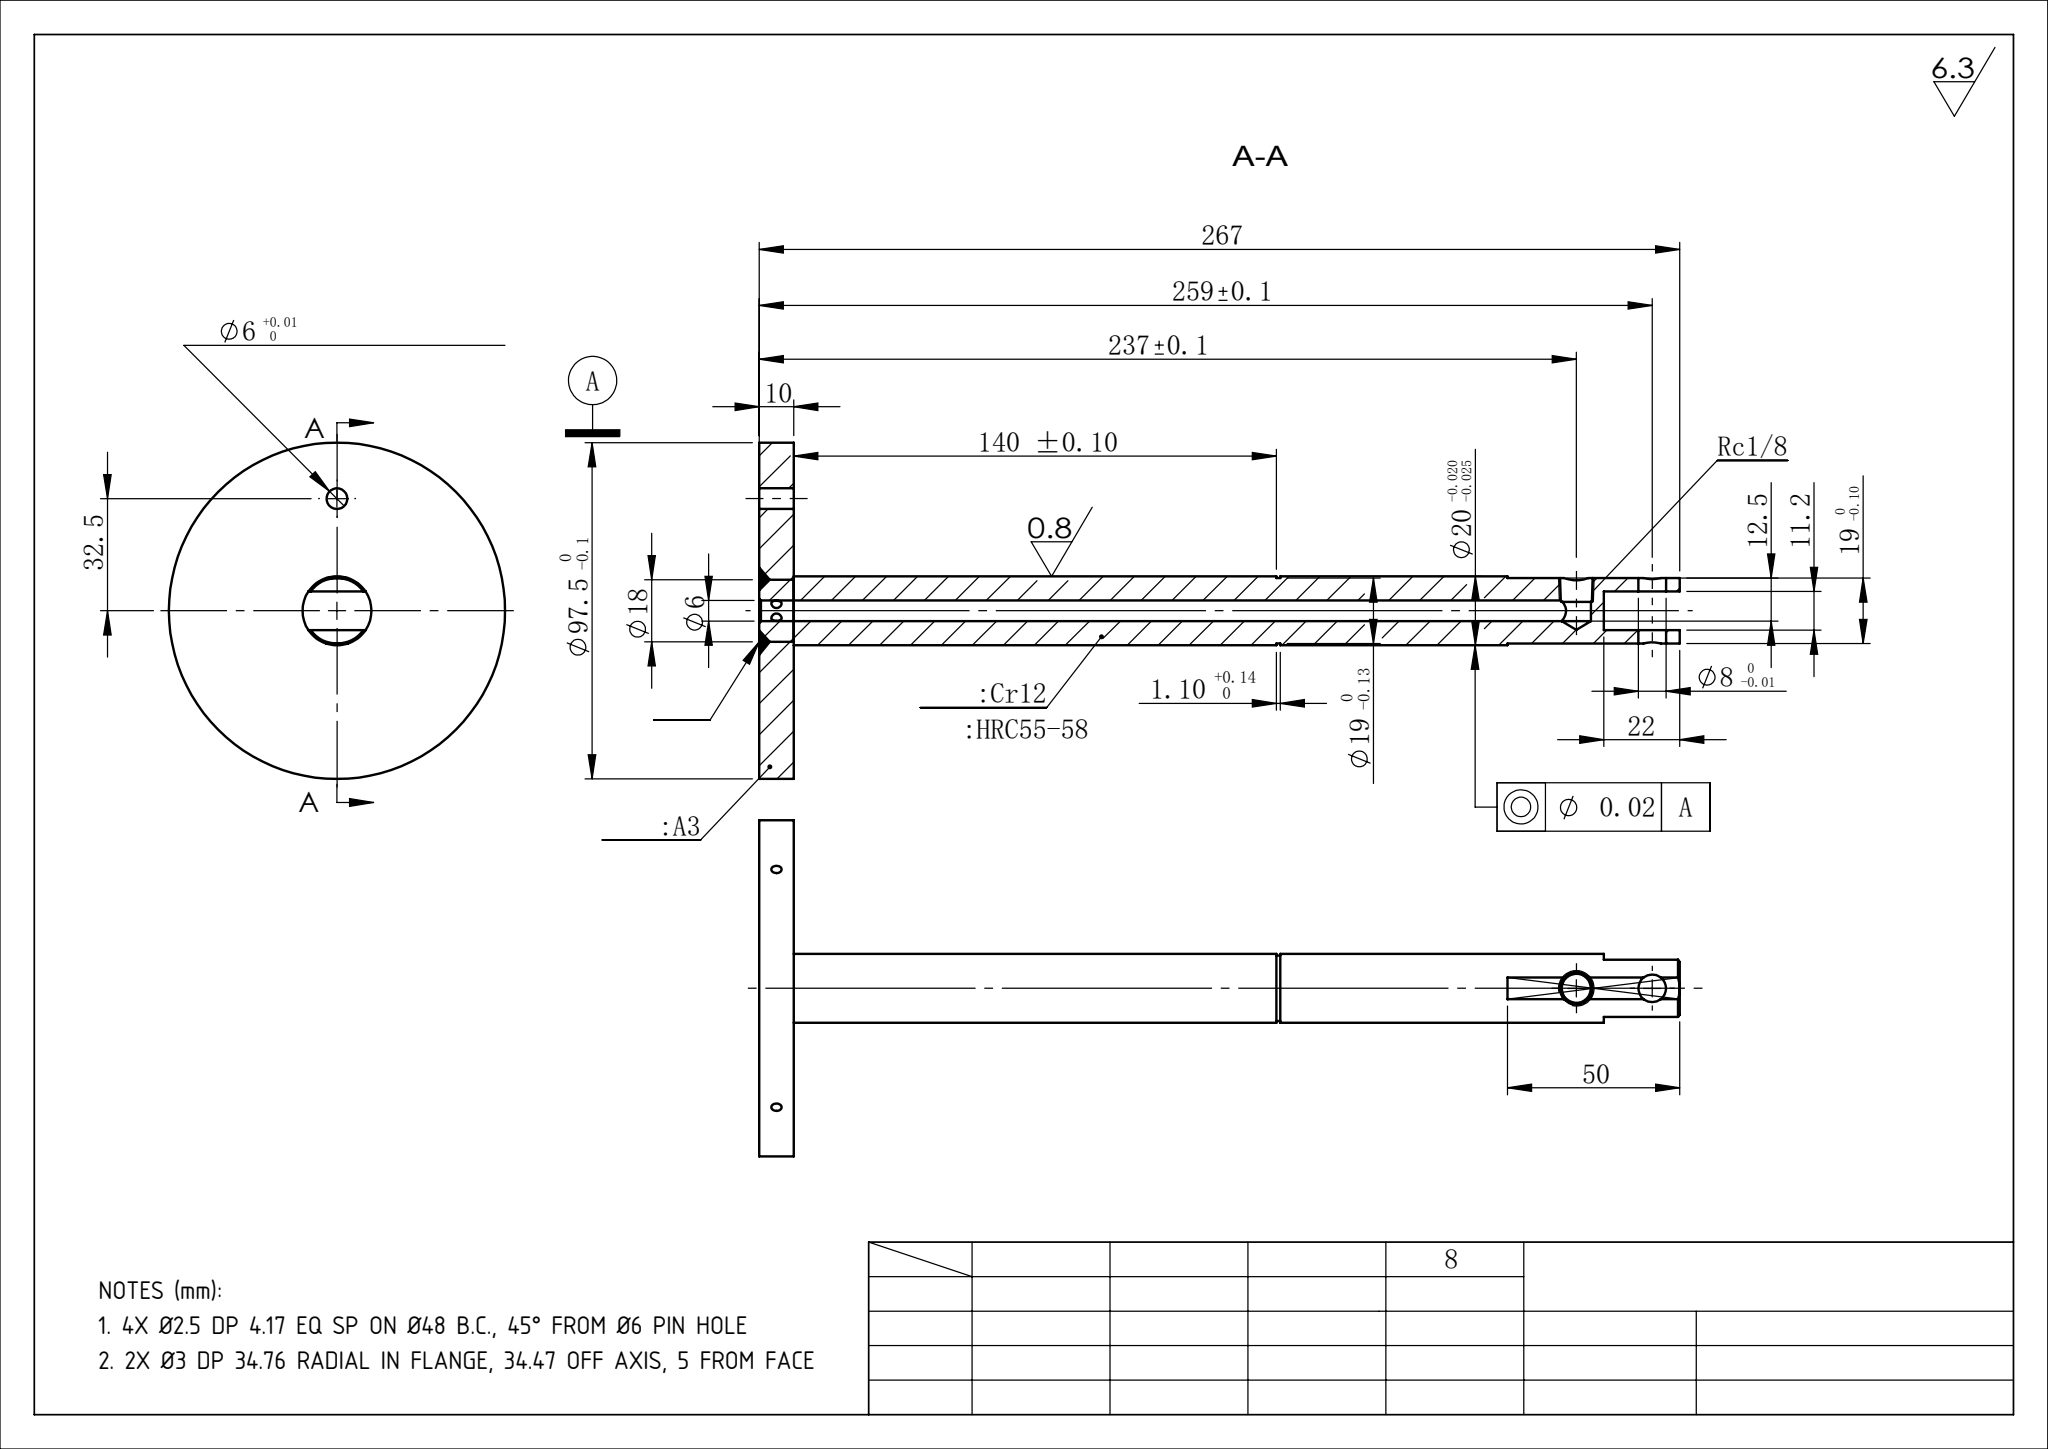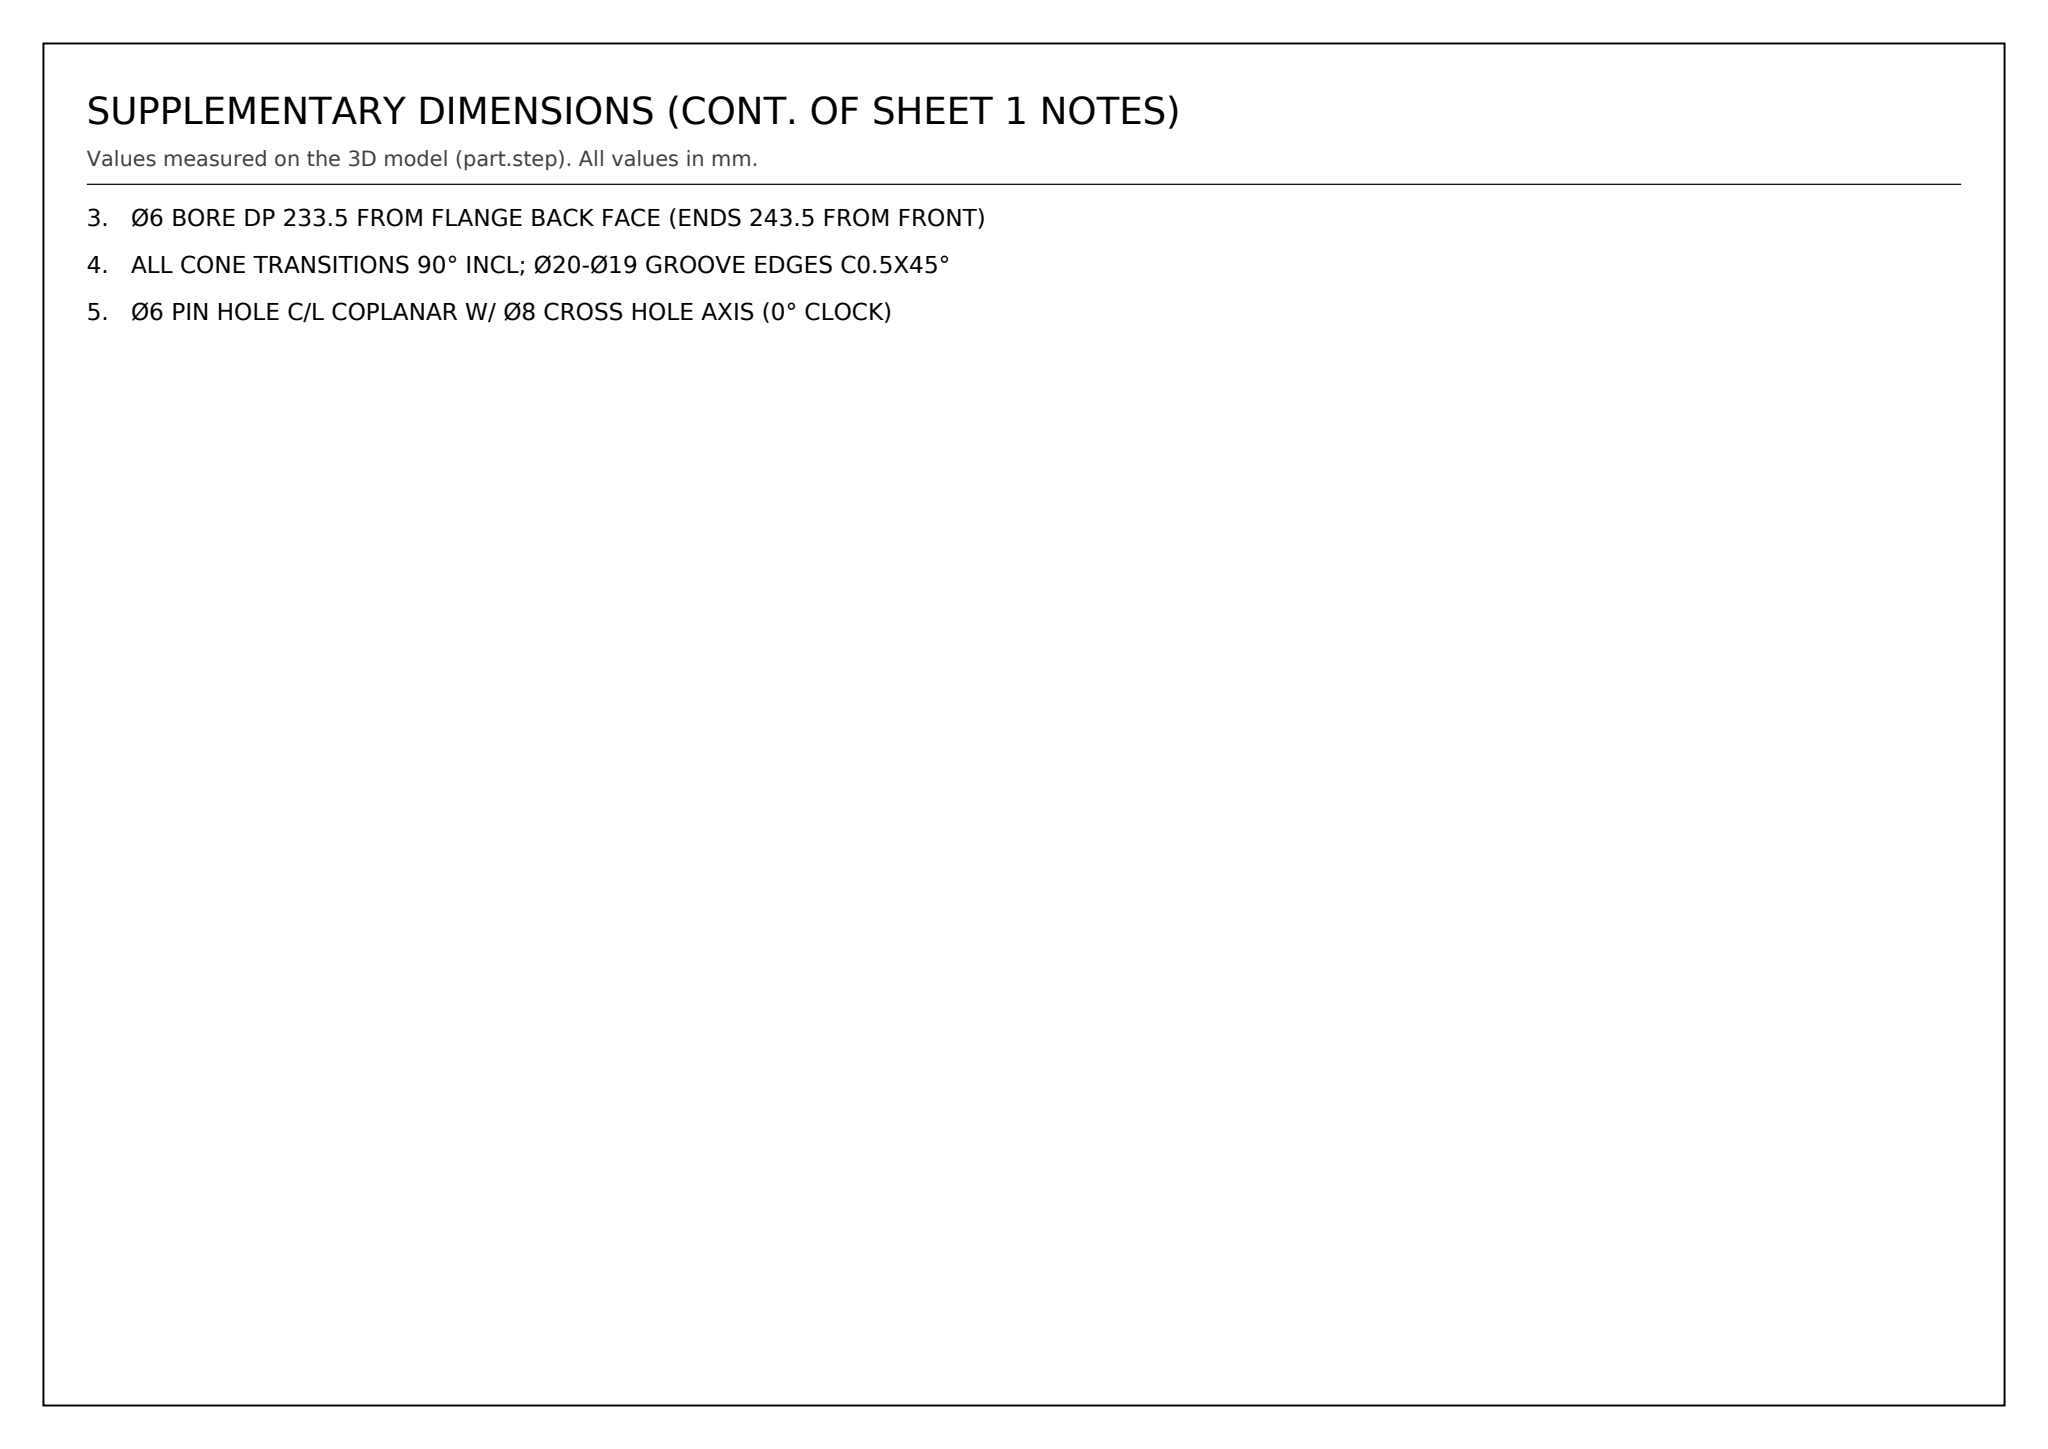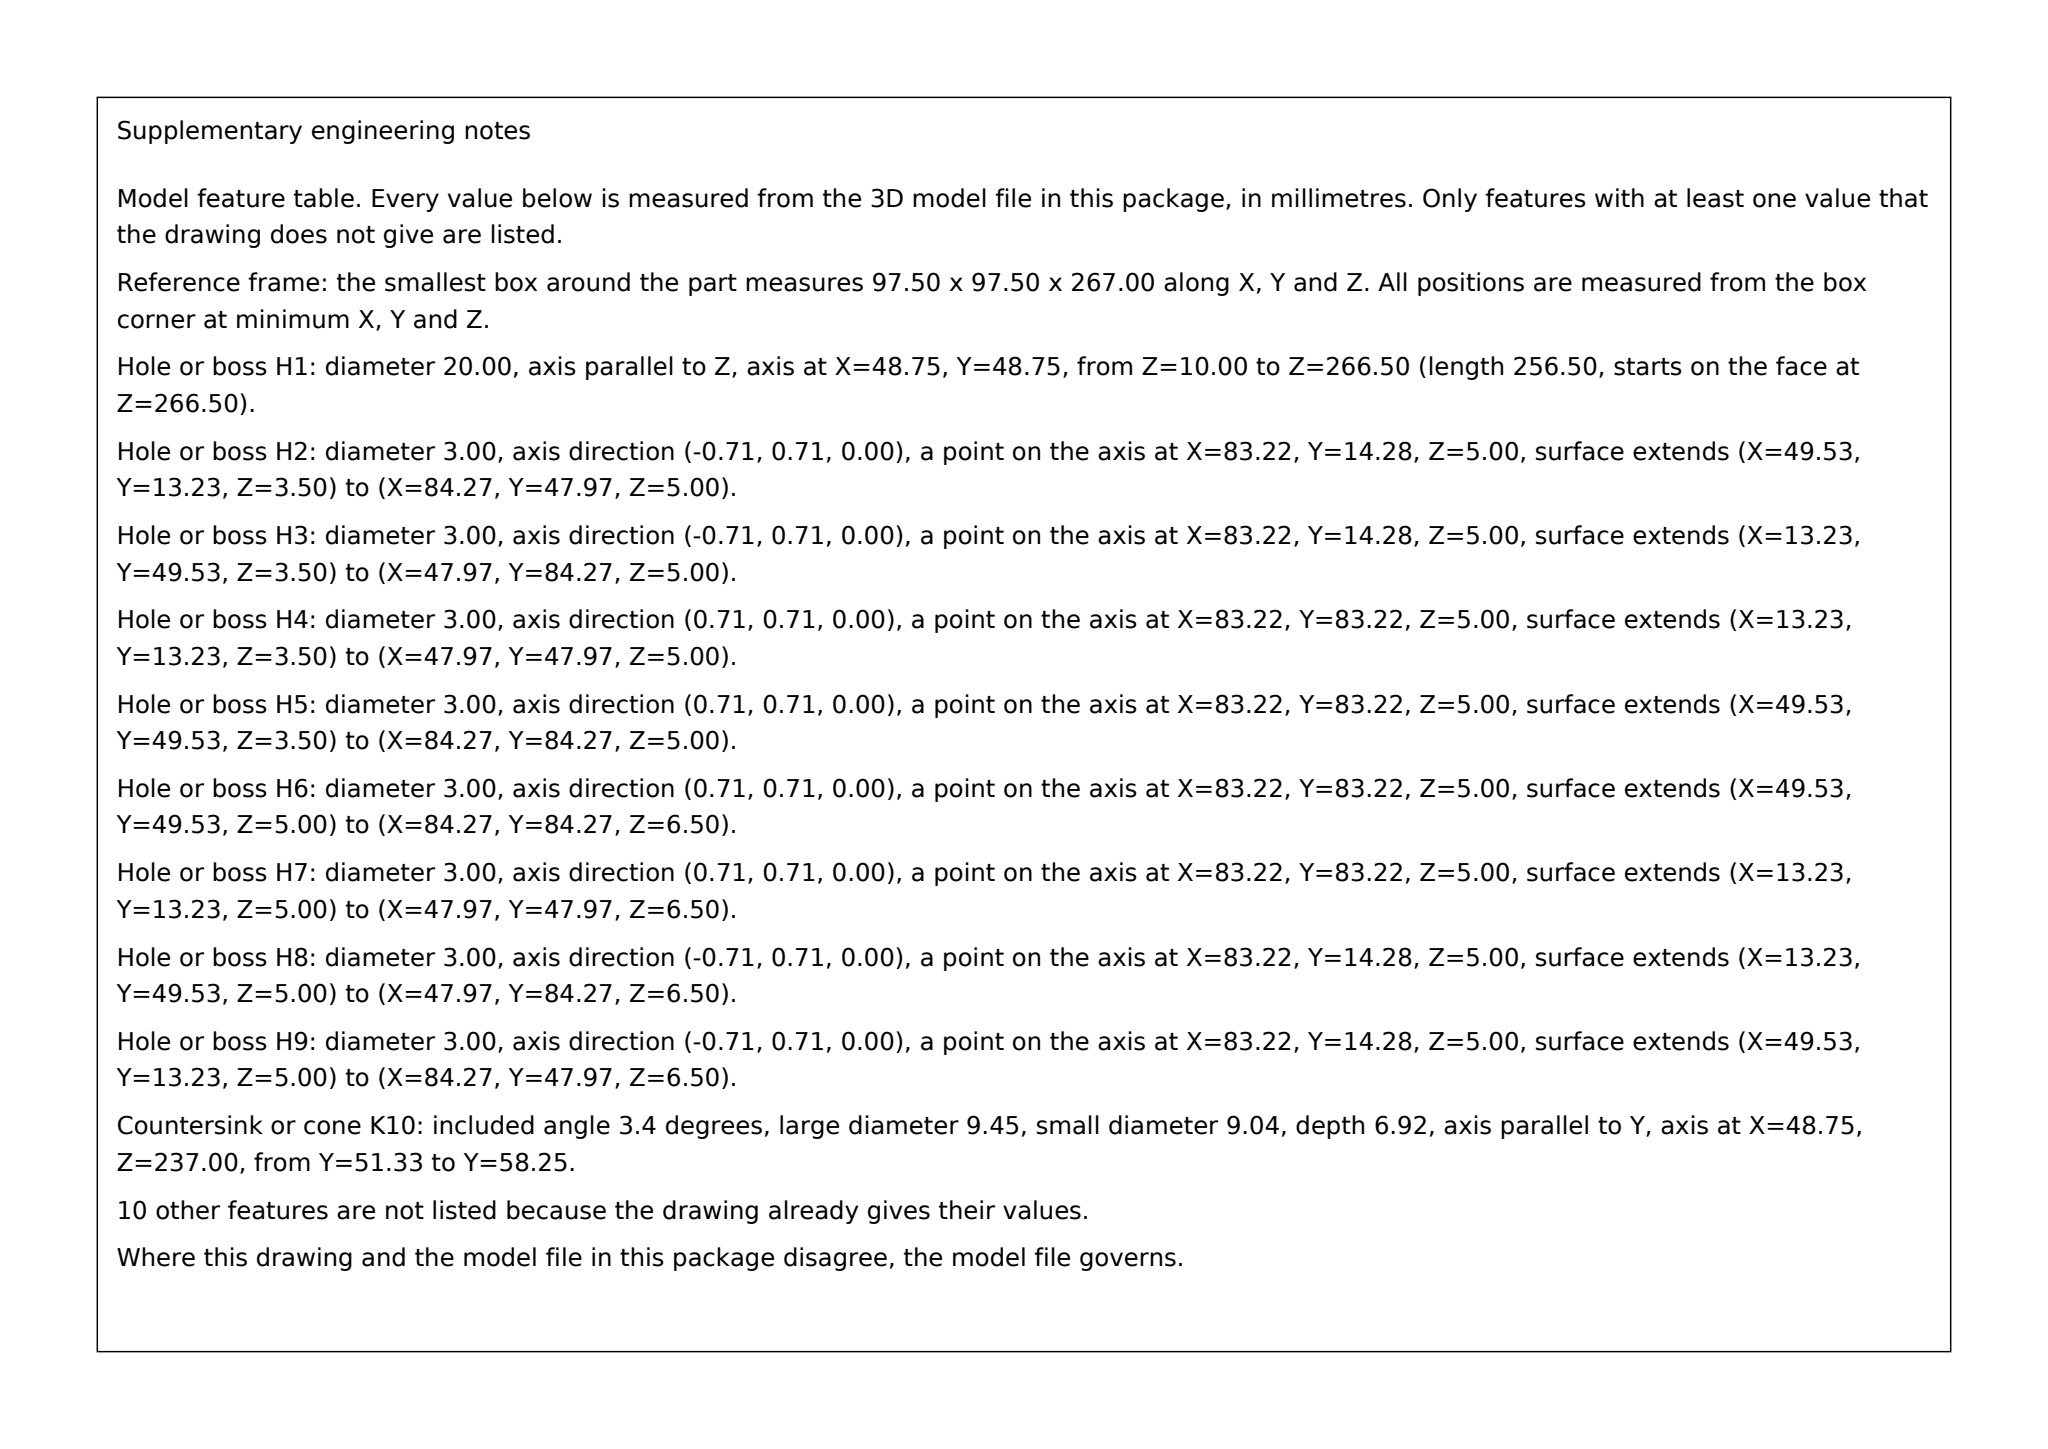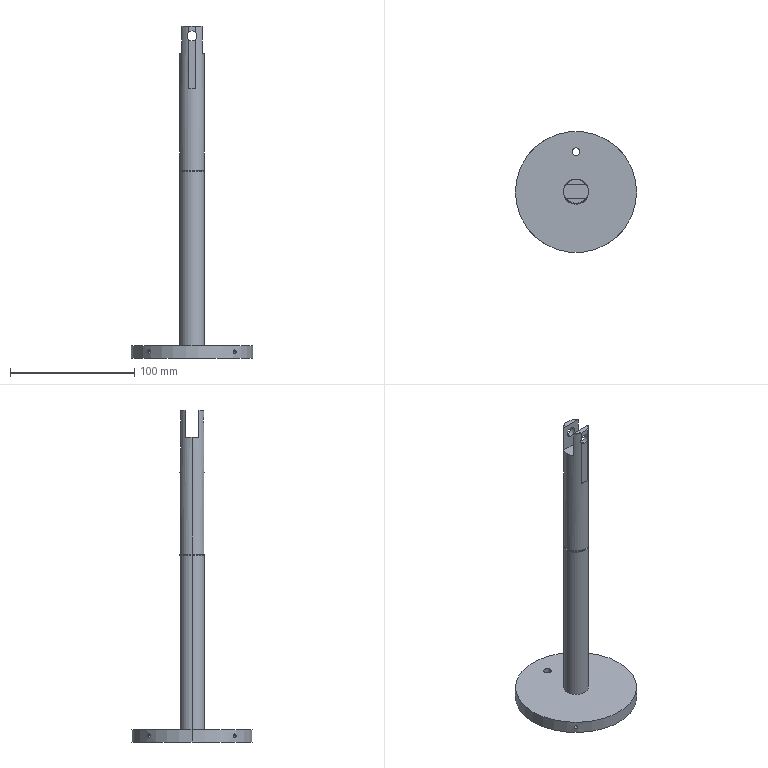Part | SolidWorks | mm | 1 solid | 61 faces | box 97.5 x 97.5 x 267 mm | volume 141042 mm3 | cylinder 34 | plane 17 | cone 10 | commonest cylinder face diameters 2.5 x8 3 x8 6 x4 20 x4 8 x4 97.5 x2 19 x2 8.433 x2
Drawing notes:
4X Ø2.5 DP 4.17 EQ SP ON Ø48 B.C., 45° FROM Ø6 PIN HOLE | from the solid: Ø2.5 z-holes at (31.78,31.78),(31.78,65.72),(65.72,31.78),(65.72,65.72); axis 48.75,48.75 -> ±16.97 diag = Ø48 B.C.; length 4.17
2X Ø3 DP 34.76 RADIAL IN FLANGE, 34.47 OFF AXIS, 5 FROM FACE | from the solid: Ø3 x-axis holes at y=14.28 & 83.22 (=48.75∓34.47), z=5, length 34.76
Ø6 BORE DP 233.5 FROM FLANGE BACK FACE (ENDS 243.5 FROM FRONT) | from the solid: Ø6 z-cyl at axis, length 233.54, starts at flange back face z=10, ends z=243.54
ALL CONE TRANSITIONS 90° INCL; Ø20-Ø19 GROOVE EDGES C0.5X45° | from the solid: cones [90.0, ref_dia 19, qty 4] and [90.0, ref_dia 6, qty 2]; Ø20->Ø19 = 0.5 radial drop
Ø6 PIN HOLE C/L COPLANAR W/ Ø8 CROSS HOLE AXIS (0° CLOCK) | from the solid: Ø6 flange hole at (48.75,81.25) = +Y 32.5; Ø8 cross holes axis = Y at z=259
build123d program:
from build123d import *

# Parameters (mm, degrees)
SKETCH1_R          = 48.75
EXTRUDE1_DEPTH     = 10
SKETCH2_R          = 10
EXTRUDE2_DEPTH     = 257
SKETCH3_W          = 33.788
SKETCH3_H          = 11.2
CUT_EXTRUDE1_DEPTH = 22
CHAMFER2_SIZE      = 0.5
SKETCH4_W          = 36.97
SKETCH4_H          = 6.667
SKETCH4_W_2        = 35.758
SKETCH4_H_2        = 6.818
CUT_EXTRUDE2_DEPTH = 50
SKETCH5_R          = 4
CUT_EXTRUDE3_DEPTH = 278.594
SKETCH8_W          = 5
SKETCH8_H          = 1.1
SKETCH9_R          = 3
CUT_EXTRUDE4_DEPTH = 236.568
CHAMFER1_SIZE      = 0.5
SKETCH10_R         = 3
CUT_EXTRUDE5_DEPTH = 276.757
SKETCH12_W         = 113.584
SKETCH12_H         = 1.5
SKETCH13_W         = 112.217
SKETCH13_H         = 1.5
SKETCH14_R         = 1.25
CUT_EXTRUDE7_DEPTH = 5


with BuildPart() as part:
    # Sketch1 → Extrude1 (new body)
    with BuildSketch(Plane.XY):
        Circle(SKETCH1_R)
    extrude(amount=EXTRUDE1_DEPTH)

    # Sketch2 → Extrude2 (add)
    with BuildSketch(Plane.XY.offset(10)):
        Circle(SKETCH2_R)
    extrude(amount=EXTRUDE2_DEPTH)

    # Sketch3 → Cut-Extrude1 (cut)
    with BuildSketch(Plane.XY.offset(267)):
        with Locations((1.212, 0)):
            Rectangle(SKETCH3_W, SKETCH3_H)
    extrude(amount=-CUT_EXTRUDE1_DEPTH, mode=Mode.SUBTRACT)

    # Chamfer2
    chamfer2_edges = [part.edges().sort_by_distance(p)[0] for p in [
        (0, -10, 267),
        (0, 10, 267),
    ]]
    chamfer(chamfer2_edges, length=CHAMFER2_SIZE)

    # Sketch4 → Cut-Extrude2 (cut)
    with BuildSketch(Plane.XY.offset(267)):
        with Locations((5.227, 12.833)):
            Rectangle(SKETCH4_W, SKETCH4_H)
        with Locations((-0.5303, -12.909)):
            Rectangle(SKETCH4_W_2, SKETCH4_H_2)
    extrude(amount=-CUT_EXTRUDE2_DEPTH, mode=Mode.SUBTRACT)

    # Sketch5 → Cut-Extrude3 (cut, through all)
    with BuildSketch(Plane(origin=(0, 9.5, 0), x_dir=(1, 0, 0), z_dir=(0, 1, 0))):
        with Locations(Location((0, -259, 0), (0, 0, 321.318))):
            Circle(SKETCH5_R)
    extrude(amount=-CUT_EXTRUDE3_DEPTH, mode=Mode.SUBTRACT)

    # Sketch7 → 1_8 NPT Tapped Hole1 (revolve, cut)
    with BuildSketch(Plane(origin=(0, 9.5, 237), x_dir=(0, 0, 1), z_dir=(1, 0, 0))):
        Polygon((0, 0), (0, 15.033), (4.216, 12.5), (4.216, 6.92), (4.537, 6.92), (4.745, 0), align=None)
    revolve(axis=Axis((0, 15.85, 237), (0, -1, 0)), mode=Mode.SUBTRACT)

    # Sketch8 → Cut-Revolve1 (revolve, cut)
    with BuildSketch(Plane(origin=(0, 0, 0), x_dir=(1, 0, 0), z_dir=(0, 1, 0)), mode=Mode.PRIVATE) as cut_revolve1_sk:
        with Locations((12, -150.55)):
            Rectangle(SKETCH8_W, SKETCH8_H)
    revolve(cut_revolve1_sk.sketch.rotate(Axis((0, 0, 0), (0, 0, 1)), 180), axis=Axis((0, 0, 0), (0, 0, 1)), mode=Mode.SUBTRACT)

    # Sketch9 → Cut-Extrude4 (cut)
    with BuildSketch(Plane(origin=(0, 0, 0), x_dir=(-1, 0, 0), z_dir=(0, 0, -1))):
        Circle(SKETCH9_R)
    extrude(amount=-CUT_EXTRUDE4_DEPTH, mode=Mode.SUBTRACT)

    # Chamfer1
    chamfer1_edges = [part.edges().sort_by_distance(p)[0] for p in [
        (3, 0, 0),
    ]]
    chamfer(chamfer1_edges, length=CHAMFER1_SIZE)

    # Sketch10 → Cut-Extrude5 (cut, through all)
    with BuildSketch(Plane(origin=(0, 0, 0), x_dir=(-1, 0, 0), z_dir=(0, 0, -1))):
        with Locations((0, 32.5)):
            Circle(SKETCH10_R)
    extrude(amount=-CUT_EXTRUDE5_DEPTH, mode=Mode.SUBTRACT)

    # Sketch12 → Cut-Revolve2 (revolve, cut)
    with BuildSketch(Plane(origin=(0, 0, 0), x_dir=(0.7071, 0.7071, 0), z_dir=(0.7071, -0.7071, 0)), mode=Mode.PRIVATE) as cut_revolve2_sk:
        with Locations((-0.2362, 5.75)):
            Rectangle(SKETCH12_W, SKETCH12_H)
    revolve(cut_revolve2_sk.sketch.rotate(Axis((34.471, 34.471, 5), (-0.7071, -0.7071, 0)), 90), axis=Axis((34.471, 34.471, 5), (-0.7071, -0.7071, 0)), mode=Mode.SUBTRACT)

    # Sketch13 → Cut-Revolve3 (revolve, cut)
    with BuildSketch(Plane(origin=(0, 0, 0), x_dir=(-0.7071, 0.7071, 0), z_dir=(0.7071, 0.7071, 0)), mode=Mode.PRIVATE) as cut_revolve3_sk:
        with Locations((0.8037, 5.75)):
            Rectangle(SKETCH13_W, SKETCH13_H)
    revolve(cut_revolve3_sk.sketch.rotate(Axis((34.471, -34.471, 5), (0.7071, -0.7071, 0)), 90), axis=Axis((34.471, -34.471, 5), (0.7071, -0.7071, 0)), mode=Mode.SUBTRACT)

    # Sketch14 → Cut-Extrude7 (cut)
    with BuildSketch(Plane(origin=(0, 0, 0), x_dir=(-1, 0, 0), z_dir=(0, 0, -1))):
        with Locations((-16.971, 16.971)):
            Circle(SKETCH14_R)
        with Locations((16.971, 16.971)):
            Circle(SKETCH14_R)
        with Locations((16.971, -16.971)):
            Circle(SKETCH14_R)
        with Locations((-16.971, -16.971)):
            Circle(SKETCH14_R)
    extrude(amount=-CUT_EXTRUDE7_DEPTH, mode=Mode.SUBTRACT)


solid = part.part